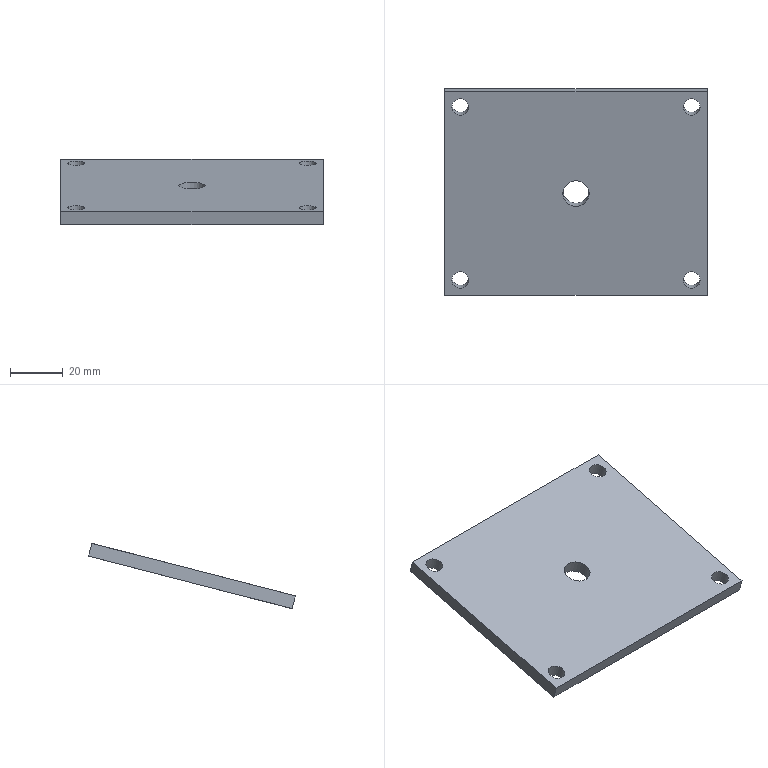Component | NX | SHIKONGGAI | 1 solid | 11 faces | box 100 x 78.71 x 24.84 mm | volume 38944 mm3 | plane 6 | cylinder 5 | commonest cylinder face diameters 6.5 x4 10 x1
STEP:
#1=CARTESIAN_POINT('',(0.,0.,0.));
#2=DIRECTION('',(0.,0.,1.));
#3=DIRECTION('',(1.,0.,0.));
#4=AXIS2_PLACEMENT_3D('',#1,#2,#3);
#5=CARTESIAN_POINT('',(-50.,133.02,11.412));
#6=VERTEX_POINT('',#5);
#7=CARTESIAN_POINT('',(-50.,55.56,-8.588));
#8=VERTEX_POINT('',#7);
#9=CARTESIAN_POINT('',(-50.,133.02,11.412));
#10=DIRECTION('',(0.,-0.9682,-0.25));
#11=VECTOR('',#10,1.);
#12=LINE('',#9,#11);
#13=CARTESIAN_POINT('',(-50.,131.77,16.253));
#14=DIRECTION('',(1.,0.,0.));
#15=DIRECTION('',(0.,0.25,-0.9682));
#16=AXIS2_PLACEMENT_3D('',#13,#14,#15);
#17=PLANE('',#16);
#18=CARTESIAN_POINT('',(5.,0.));
#19=DIRECTION('',(0.,-1.));
#20=VECTOR('',#19,1.);
#21=LINE('',#18,#20);
#22=(GEOMETRIC_REPRESENTATION_CONTEXT(2)PARAMETRIC_REPRESENTATION_CONTEXT()REPRESENTATION_CONTEXT('',''));
#23=DEFINITIONAL_REPRESENTATION('',(#21),#22);
#24=PCURVE('',#17,#23);
#25=CARTESIAN_POINT('',(44.,127.211,9.912));
#26=DIRECTION('',(0.,0.25,-0.9682));
#27=DIRECTION('',(-1.,0.,0.));
#28=AXIS2_PLACEMENT_3D('',#25,#26,#27);
#29=PLANE('',#28);
#30=CARTESIAN_POINT('',(94.,6.));
#31=DIRECTION('',(0.,-1.));
#32=VECTOR('',#31,1.);
#33=LINE('',#30,#32);
#34=(GEOMETRIC_REPRESENTATION_CONTEXT(2)PARAMETRIC_REPRESENTATION_CONTEXT()REPRESENTATION_CONTEXT('',''));
#35=DEFINITIONAL_REPRESENTATION('',(#33),#34);
#36=PCURVE('',#29,#35);
#37=SURFACE_CURVE('',#12,(#24,#36),.PCURVE_S1.);
#38=EDGE_CURVE('',#6,#8,#37,.T.);
#39=ORIENTED_EDGE('',*,*,#38,.T.);
#40=CARTESIAN_POINT('',(-50.,54.31,-3.747));
#41=VERTEX_POINT('',#40);
#42=CARTESIAN_POINT('',(-50.,54.31,-3.747));
#43=DIRECTION('',(0.,0.25,-0.9682));
#44=VECTOR('',#43,1.);
#45=LINE('',#42,#44);
#46=CARTESIAN_POINT('',(-0.,-80.));
#47=DIRECTION('',(1.,0.));
#48=VECTOR('',#47,1.);
#49=LINE('',#46,#48);
#50=(GEOMETRIC_REPRESENTATION_CONTEXT(2)PARAMETRIC_REPRESENTATION_CONTEXT()REPRESENTATION_CONTEXT('',''));
#51=DEFINITIONAL_REPRESENTATION('',(#49),#50);
#52=PCURVE('',#17,#51);
#53=CARTESIAN_POINT('',(-50.,54.31,-3.747));
#54=DIRECTION('',(0.,0.9682,0.25));
#55=DIRECTION('',(0.,-0.25,0.9682));
#56=AXIS2_PLACEMENT_3D('',#53,#54,#55);
#57=PLANE('',#56);
#58=CARTESIAN_POINT('',(0.,0.));
#59=DIRECTION('',(-1.,0.));
#60=VECTOR('',#59,1.);
#61=LINE('',#58,#60);
#62=(GEOMETRIC_REPRESENTATION_CONTEXT(2)PARAMETRIC_REPRESENTATION_CONTEXT()REPRESENTATION_CONTEXT('',''));
#63=DEFINITIONAL_REPRESENTATION('',(#61),#62);
#64=PCURVE('',#57,#63);
#65=SURFACE_CURVE('',#45,(#52,#64),.PCURVE_S1.);
#66=EDGE_CURVE('',#41,#8,#65,.T.);
#67=ORIENTED_EDGE('',*,*,#66,.F.);
#68=CARTESIAN_POINT('',(-50.,131.77,16.253));
#69=VERTEX_POINT('',#68);
#70=CARTESIAN_POINT('',(-50.,131.77,16.253));
#71=DIRECTION('',(0.,-0.9682,-0.25));
#72=VECTOR('',#71,1.);
#73=LINE('',#70,#72);
#74=CARTESIAN_POINT('',(0.,0.));
#75=DIRECTION('',(0.,-1.));
#76=VECTOR('',#75,1.);
#77=LINE('',#74,#76);
#78=(GEOMETRIC_REPRESENTATION_CONTEXT(2)PARAMETRIC_REPRESENTATION_CONTEXT()REPRESENTATION_CONTEXT('',''));
#79=DEFINITIONAL_REPRESENTATION('',(#77),#78);
#80=PCURVE('',#17,#79);
#81=CARTESIAN_POINT('',(44.,125.961,14.753));
#82=DIRECTION('',(0.,0.25,-0.9682));
#83=DIRECTION('',(-1.,0.,0.));
#84=AXIS2_PLACEMENT_3D('',#81,#82,#83);
#85=PLANE('',#84);
#86=CARTESIAN_POINT('',(94.,6.));
#87=DIRECTION('',(0.,-1.));
#88=VECTOR('',#87,1.);
#89=LINE('',#86,#88);
#90=(GEOMETRIC_REPRESENTATION_CONTEXT(2)PARAMETRIC_REPRESENTATION_CONTEXT()REPRESENTATION_CONTEXT('',''));
#91=DEFINITIONAL_REPRESENTATION('',(#89),#90);
#92=PCURVE('',#85,#91);
#93=SURFACE_CURVE('',#73,(#80,#92),.PCURVE_S1.);
#94=EDGE_CURVE('',#69,#41,#93,.T.);
#95=ORIENTED_EDGE('',*,*,#94,.F.);
#96=CARTESIAN_POINT('',(-50.,131.77,16.253));
#97=DIRECTION('',(0.,0.25,-0.9682));
#98=VECTOR('',#97,1.);
#99=LINE('',#96,#98);
#100=CARTESIAN_POINT('',(0.,0.));
#101=DIRECTION('',(1.,0.));
#102=VECTOR('',#101,1.);
#103=LINE('',#100,#102);
#104=(GEOMETRIC_REPRESENTATION_CONTEXT(2)PARAMETRIC_REPRESENTATION_CONTEXT()REPRESENTATION_CONTEXT('',''));
#105=DEFINITIONAL_REPRESENTATION('',(#103),#104);
#106=PCURVE('',#17,#105);
#107=CARTESIAN_POINT('',(50.,131.77,16.253));
#108=DIRECTION('',(0.,-0.9682,-0.25));
#109=DIRECTION('',(0.,0.25,-0.9682));
#110=AXIS2_PLACEMENT_3D('',#107,#108,#109);
#111=PLANE('',#110);
#112=CARTESIAN_POINT('',(0.,-100.));
#113=DIRECTION('',(1.,0.));
#114=VECTOR('',#113,1.);
#115=LINE('',#112,#114);
#116=(GEOMETRIC_REPRESENTATION_CONTEXT(2)PARAMETRIC_REPRESENTATION_CONTEXT()REPRESENTATION_CONTEXT('',''));
#117=DEFINITIONAL_REPRESENTATION('',(#115),#116);
#118=PCURVE('',#111,#117);
#119=SURFACE_CURVE('',#99,(#106,#118),.PCURVE_S1.);
#120=EDGE_CURVE('',#69,#6,#119,.T.);
#121=ORIENTED_EDGE('',*,*,#120,.T.);
#122=EDGE_LOOP('',(#39,#67,#95,#121));
#123=FACE_BOUND('',#122,.T.);
#124=ADVANCED_FACE('',(#123),#17,.F.);
#125=CARTESIAN_POINT('',(50.,55.56,-8.588));
#126=VERTEX_POINT('',#125);
#127=CARTESIAN_POINT('',(-50.,55.56,-8.588));
#128=DIRECTION('',(1.,0.,0.));
#129=VECTOR('',#128,1.);
#130=LINE('',#127,#129);
#131=CARTESIAN_POINT('',(-5.,0.));
#132=DIRECTION('',(0.,1.));
#133=VECTOR('',#132,1.);
#134=LINE('',#131,#133);
#135=(GEOMETRIC_REPRESENTATION_CONTEXT(2)PARAMETRIC_REPRESENTATION_CONTEXT()REPRESENTATION_CONTEXT('',''));
#136=DEFINITIONAL_REPRESENTATION('',(#134),#135);
#137=PCURVE('',#57,#136);
#138=CARTESIAN_POINT('',(94.,-74.));
#139=DIRECTION('',(-1.,0.));
#140=VECTOR('',#139,1.);
#141=LINE('',#138,#140);
#142=(GEOMETRIC_REPRESENTATION_CONTEXT(2)PARAMETRIC_REPRESENTATION_CONTEXT()REPRESENTATION_CONTEXT('',''));
#143=DEFINITIONAL_REPRESENTATION('',(#141),#142);
#144=PCURVE('',#29,#143);
#145=SURFACE_CURVE('',#130,(#137,#144),.PCURVE_S1.);
#146=EDGE_CURVE('',#8,#126,#145,.T.);
#147=ORIENTED_EDGE('',*,*,#146,.T.);
#148=CARTESIAN_POINT('',(50.,54.31,-3.747));
#149=VERTEX_POINT('',#148);
#150=CARTESIAN_POINT('',(50.,54.31,-3.747));
#151=DIRECTION('',(0.,0.25,-0.9682));
#152=VECTOR('',#151,1.);
#153=LINE('',#150,#152);
#154=CARTESIAN_POINT('',(0.,100.));
#155=DIRECTION('',(-1.,0.));
#156=VECTOR('',#155,1.);
#157=LINE('',#154,#156);
#158=(GEOMETRIC_REPRESENTATION_CONTEXT(2)PARAMETRIC_REPRESENTATION_CONTEXT()REPRESENTATION_CONTEXT('',''));
#159=DEFINITIONAL_REPRESENTATION('',(#157),#158);
#160=PCURVE('',#57,#159);
#161=CARTESIAN_POINT('',(50.,54.31,-3.747));
#162=DIRECTION('',(-1.,0.,0.));
#163=DIRECTION('',(0.,-0.25,0.9682));
#164=AXIS2_PLACEMENT_3D('',#161,#162,#163);
#165=PLANE('',#164);
#166=CARTESIAN_POINT('',(0.,0.));
#167=DIRECTION('',(-1.,0.));
#168=VECTOR('',#167,1.);
#169=LINE('',#166,#168);
#170=(GEOMETRIC_REPRESENTATION_CONTEXT(2)PARAMETRIC_REPRESENTATION_CONTEXT()REPRESENTATION_CONTEXT('',''));
#171=DEFINITIONAL_REPRESENTATION('',(#169),#170);
#172=PCURVE('',#165,#171);
#173=SURFACE_CURVE('',#153,(#160,#172),.PCURVE_S1.);
#174=EDGE_CURVE('',#149,#126,#173,.T.);
#175=ORIENTED_EDGE('',*,*,#174,.F.);
#176=CARTESIAN_POINT('',(-50.,54.31,-3.747));
#177=DIRECTION('',(1.,0.,0.));
#178=VECTOR('',#177,1.);
#179=LINE('',#176,#178);
#180=CARTESIAN_POINT('',(0.,0.));
#181=DIRECTION('',(0.,1.));
#182=VECTOR('',#181,1.);
#183=LINE('',#180,#182);
#184=(GEOMETRIC_REPRESENTATION_CONTEXT(2)PARAMETRIC_REPRESENTATION_CONTEXT()REPRESENTATION_CONTEXT('',''));
#185=DEFINITIONAL_REPRESENTATION('',(#183),#184);
#186=PCURVE('',#57,#185);
#187=CARTESIAN_POINT('',(94.,-74.));
#188=DIRECTION('',(-1.,0.));
#189=VECTOR('',#188,1.);
#190=LINE('',#187,#189);
#191=(GEOMETRIC_REPRESENTATION_CONTEXT(2)PARAMETRIC_REPRESENTATION_CONTEXT()REPRESENTATION_CONTEXT('',''));
#192=DEFINITIONAL_REPRESENTATION('',(#190),#191);
#193=PCURVE('',#85,#192);
#194=SURFACE_CURVE('',#179,(#186,#193),.PCURVE_S1.);
#195=EDGE_CURVE('',#41,#149,#194,.T.);
#196=ORIENTED_EDGE('',*,*,#195,.F.);
#197=ORIENTED_EDGE('',*,*,#66,.T.);
#198=EDGE_LOOP('',(#147,#175,#196,#197));
#199=FACE_BOUND('',#198,.T.);
#200=ADVANCED_FACE('',(#199),#57,.F.);
#201=CARTESIAN_POINT('',(50.,133.02,11.412));
#202=VERTEX_POINT('',#201);
#203=CARTESIAN_POINT('',(50.,55.56,-8.588));
#204=DIRECTION('',(0.,0.9682,0.25));
#205=VECTOR('',#204,1.);
#206=LINE('',#203,#205);
#207=CARTESIAN_POINT('',(-5.,0.));
#208=DIRECTION('',(0.,1.));
#209=VECTOR('',#208,1.);
#210=LINE('',#207,#209);
#211=(GEOMETRIC_REPRESENTATION_CONTEXT(2)PARAMETRIC_REPRESENTATION_CONTEXT()REPRESENTATION_CONTEXT('',''));
#212=DEFINITIONAL_REPRESENTATION('',(#210),#211);
#213=PCURVE('',#165,#212);
#214=CARTESIAN_POINT('',(-6.,-74.));
#215=DIRECTION('',(0.,1.));
#216=VECTOR('',#215,1.);
#217=LINE('',#214,#216);
#218=(GEOMETRIC_REPRESENTATION_CONTEXT(2)PARAMETRIC_REPRESENTATION_CONTEXT()REPRESENTATION_CONTEXT('',''));
#219=DEFINITIONAL_REPRESENTATION('',(#217),#218);
#220=PCURVE('',#29,#219);
#221=SURFACE_CURVE('',#206,(#213,#220),.PCURVE_S1.);
#222=EDGE_CURVE('',#126,#202,#221,.T.);
#223=ORIENTED_EDGE('',*,*,#222,.T.);
#224=CARTESIAN_POINT('',(50.,131.77,16.253));
#225=VERTEX_POINT('',#224);
#226=CARTESIAN_POINT('',(50.,131.77,16.253));
#227=DIRECTION('',(0.,0.25,-0.9682));
#228=VECTOR('',#227,1.);
#229=LINE('',#226,#228);
#230=CARTESIAN_POINT('',(-0.,80.));
#231=DIRECTION('',(-1.,0.));
#232=VECTOR('',#231,1.);
#233=LINE('',#230,#232);
#234=(GEOMETRIC_REPRESENTATION_CONTEXT(2)PARAMETRIC_REPRESENTATION_CONTEXT()REPRESENTATION_CONTEXT('',''));
#235=DEFINITIONAL_REPRESENTATION('',(#233),#234);
#236=PCURVE('',#165,#235);
#237=CARTESIAN_POINT('',(0.,0.));
#238=DIRECTION('',(1.,0.));
#239=VECTOR('',#238,1.);
#240=LINE('',#237,#239);
#241=(GEOMETRIC_REPRESENTATION_CONTEXT(2)PARAMETRIC_REPRESENTATION_CONTEXT()REPRESENTATION_CONTEXT('',''));
#242=DEFINITIONAL_REPRESENTATION('',(#240),#241);
#243=PCURVE('',#111,#242);
#244=SURFACE_CURVE('',#229,(#236,#243),.PCURVE_S1.);
#245=EDGE_CURVE('',#225,#202,#244,.T.);
#246=ORIENTED_EDGE('',*,*,#245,.F.);
#247=CARTESIAN_POINT('',(50.,54.31,-3.747));
#248=DIRECTION('',(0.,0.9682,0.25));
#249=VECTOR('',#248,1.);
#250=LINE('',#247,#249);
#251=CARTESIAN_POINT('',(0.,0.));
#252=DIRECTION('',(0.,1.));
#253=VECTOR('',#252,1.);
#254=LINE('',#251,#253);
#255=(GEOMETRIC_REPRESENTATION_CONTEXT(2)PARAMETRIC_REPRESENTATION_CONTEXT()REPRESENTATION_CONTEXT('',''));
#256=DEFINITIONAL_REPRESENTATION('',(#254),#255);
#257=PCURVE('',#165,#256);
#258=CARTESIAN_POINT('',(-6.,-74.));
#259=DIRECTION('',(0.,1.));
#260=VECTOR('',#259,1.);
#261=LINE('',#258,#260);
#262=(GEOMETRIC_REPRESENTATION_CONTEXT(2)PARAMETRIC_REPRESENTATION_CONTEXT()REPRESENTATION_CONTEXT('',''));
#263=DEFINITIONAL_REPRESENTATION('',(#261),#262);
#264=PCURVE('',#85,#263);
#265=SURFACE_CURVE('',#250,(#257,#264),.PCURVE_S1.);
#266=EDGE_CURVE('',#149,#225,#265,.T.);
#267=ORIENTED_EDGE('',*,*,#266,.F.);
#268=ORIENTED_EDGE('',*,*,#174,.T.);
#269=EDGE_LOOP('',(#223,#246,#267,#268));
#270=FACE_BOUND('',#269,.T.);
#271=ADVANCED_FACE('',(#270),#165,.F.);
#272=CARTESIAN_POINT('',(-40.75,125.961,14.753));
#273=VERTEX_POINT('',#272);
#274=CARTESIAN_POINT('',(-44.,125.961,14.753));
#275=DIRECTION('',(0.,-0.25,0.9682));
#276=DIRECTION('',(1.,0.,0.));
#277=AXIS2_PLACEMENT_3D('',#274,#275,#276);
#278=CIRCLE('',#277,3.25);
#279=CARTESIAN_POINT('',(-44.,125.961,14.753));
#280=DIRECTION('',(0.,0.25,-0.9682));
#281=DIRECTION('',(-1.,0.,0.));
#282=AXIS2_PLACEMENT_3D('',#279,#280,#281);
#283=CYLINDRICAL_SURFACE('',#282,3.25);
#284=CARTESIAN_POINT('',(9.425,0.));
#285=DIRECTION('',(-1.,0.));
#286=VECTOR('',#285,1.);
#287=LINE('',#284,#286);
#288=(GEOMETRIC_REPRESENTATION_CONTEXT(2)PARAMETRIC_REPRESENTATION_CONTEXT()REPRESENTATION_CONTEXT('',''));
#289=DEFINITIONAL_REPRESENTATION('',(#287),#288);
#290=PCURVE('',#283,#289);
#291=CARTESIAN_POINT('',(84.75,0.));
#292=CARTESIAN_POINT('',(84.75,5.629));
#293=CARTESIAN_POINT('',(89.625,2.815));
#294=CARTESIAN_POINT('',(94.5,0.));
#295=CARTESIAN_POINT('',(89.625,-2.815));
#296=CARTESIAN_POINT('',(84.75,-5.629));
#297=CARTESIAN_POINT('',(84.75,0.));
#298=(BOUNDED_CURVE()B_SPLINE_CURVE(2,(#291,#292,#293,#294,#295,#296,#297),.UNSPECIFIED.,.T.,.F.)B_SPLINE_CURVE_WITH_KNOTS((1,2,2,2,2,1),(-2.094,0.,2.094,4.189,6.283,8.378),.UNSPECIFIED.)CURVE()GEOMETRIC_REPRESENTATION_ITEM()RATIONAL_B_SPLINE_CURVE((1.,0.5,1.,0.5,1.,0.5,1.))REPRESENTATION_ITEM(''));
#299=(GEOMETRIC_REPRESENTATION_CONTEXT(2)PARAMETRIC_REPRESENTATION_CONTEXT()REPRESENTATION_CONTEXT('',''));
#300=DEFINITIONAL_REPRESENTATION('',(#298),#299);
#301=PCURVE('',#85,#300);
#302=SURFACE_CURVE('',#278,(#290,#301),.PCURVE_S1.);
#303=EDGE_CURVE('',#273,#273,#302,.T.);
#304=ORIENTED_EDGE('',*,*,#303,.F.);
#305=CARTESIAN_POINT('',(-40.75,127.211,9.912));
#306=VERTEX_POINT('',#305);
#307=CARTESIAN_POINT('',(-40.75,125.961,14.753));
#308=CARTESIAN_POINT('',(-40.75,127.211,9.912));
#309=B_SPLINE_CURVE_WITH_KNOTS('',1,(#307,#308),.UNSPECIFIED.,.F.,.F.,(2,2),(0.,5.),.PIECEWISE_BEZIER_KNOTS.);
#310=CARTESIAN_POINT('',(9.425,0.));
#311=DIRECTION('',(0.,1.));
#312=VECTOR('',#311,1.);
#313=LINE('',#310,#312);
#314=(GEOMETRIC_REPRESENTATION_CONTEXT(2)PARAMETRIC_REPRESENTATION_CONTEXT()REPRESENTATION_CONTEXT('',''));
#315=DEFINITIONAL_REPRESENTATION('',(#313),#314);
#316=PCURVE('',#283,#315);
#317=CARTESIAN_POINT('',(3.142,0.));
#318=DIRECTION('',(0.,1.));
#319=VECTOR('',#318,1.);
#320=LINE('',#317,#319);
#321=(GEOMETRIC_REPRESENTATION_CONTEXT(2)PARAMETRIC_REPRESENTATION_CONTEXT()REPRESENTATION_CONTEXT('',''));
#322=DEFINITIONAL_REPRESENTATION('',(#320),#321);
#323=PCURVE('',#283,#322);
#324=SEAM_CURVE('',#309,(#316,#323),.PCURVE_S1.);
#325=EDGE_CURVE('',#273,#306,#324,.T.);
#326=ORIENTED_EDGE('',*,*,#325,.T.);
#327=CARTESIAN_POINT('',(-44.,127.211,9.912));
#328=DIRECTION('',(0.,-0.25,0.9682));
#329=DIRECTION('',(1.,0.,0.));
#330=AXIS2_PLACEMENT_3D('',#327,#328,#329);
#331=CIRCLE('',#330,3.25);
#332=CARTESIAN_POINT('',(9.425,5.));
#333=DIRECTION('',(-1.,0.));
#334=VECTOR('',#333,1.);
#335=LINE('',#332,#334);
#336=(GEOMETRIC_REPRESENTATION_CONTEXT(2)PARAMETRIC_REPRESENTATION_CONTEXT()REPRESENTATION_CONTEXT('',''));
#337=DEFINITIONAL_REPRESENTATION('',(#335),#336);
#338=PCURVE('',#283,#337);
#339=CARTESIAN_POINT('',(84.75,0.));
#340=CARTESIAN_POINT('',(84.75,5.629));
#341=CARTESIAN_POINT('',(89.625,2.815));
#342=CARTESIAN_POINT('',(94.5,0.));
#343=CARTESIAN_POINT('',(89.625,-2.815));
#344=CARTESIAN_POINT('',(84.75,-5.629));
#345=CARTESIAN_POINT('',(84.75,0.));
#346=(BOUNDED_CURVE()B_SPLINE_CURVE(2,(#339,#340,#341,#342,#343,#344,#345),.UNSPECIFIED.,.T.,.F.)B_SPLINE_CURVE_WITH_KNOTS((1,2,2,2,2,1),(-2.094,0.,2.094,4.189,6.283,8.378),.UNSPECIFIED.)CURVE()GEOMETRIC_REPRESENTATION_ITEM()RATIONAL_B_SPLINE_CURVE((1.,0.5,1.,0.5,1.,0.5,1.))REPRESENTATION_ITEM(''));
#347=(GEOMETRIC_REPRESENTATION_CONTEXT(2)PARAMETRIC_REPRESENTATION_CONTEXT()REPRESENTATION_CONTEXT('',''));
#348=DEFINITIONAL_REPRESENTATION('',(#346),#347);
#349=PCURVE('',#29,#348);
#350=SURFACE_CURVE('',#331,(#338,#349),.PCURVE_S1.);
#351=EDGE_CURVE('',#306,#306,#350,.T.);
#352=ORIENTED_EDGE('',*,*,#351,.T.);
#353=ORIENTED_EDGE('',*,*,#325,.F.);
#354=EDGE_LOOP('',(#304,#326,#352,#353));
#355=FACE_BOUND('',#354,.F.);
#356=ADVANCED_FACE('',(#355),#283,.F.);
#357=CARTESIAN_POINT('',(40.75,60.12,-2.247));
#358=VERTEX_POINT('',#357);
#359=CARTESIAN_POINT('',(44.,60.12,-2.247));
#360=DIRECTION('',(0.,-0.25,0.9682));
#361=DIRECTION('',(-1.,0.,0.));
#362=AXIS2_PLACEMENT_3D('',#359,#360,#361);
#363=CIRCLE('',#362,3.25);
#364=CARTESIAN_POINT('',(44.,60.12,-2.247));
#365=DIRECTION('',(0.,0.25,-0.9682));
#366=DIRECTION('',(-1.,0.,0.));
#367=AXIS2_PLACEMENT_3D('',#364,#365,#366);
#368=CYLINDRICAL_SURFACE('',#367,3.25);
#369=CARTESIAN_POINT('',(6.283,0.));
#370=DIRECTION('',(-1.,0.));
#371=VECTOR('',#370,1.);
#372=LINE('',#369,#371);
#373=(GEOMETRIC_REPRESENTATION_CONTEXT(2)PARAMETRIC_REPRESENTATION_CONTEXT()REPRESENTATION_CONTEXT('',''));
#374=DEFINITIONAL_REPRESENTATION('',(#372),#373);
#375=PCURVE('',#368,#374);
#376=CARTESIAN_POINT('',(3.25,-68.));
#377=CARTESIAN_POINT('',(3.25,-73.629));
#378=CARTESIAN_POINT('',(-1.625,-70.815));
#379=CARTESIAN_POINT('',(-6.5,-68.));
#380=CARTESIAN_POINT('',(-1.625,-65.185));
#381=CARTESIAN_POINT('',(3.25,-62.371));
#382=CARTESIAN_POINT('',(3.25,-68.));
#383=(BOUNDED_CURVE()B_SPLINE_CURVE(2,(#376,#377,#378,#379,#380,#381,#382),.UNSPECIFIED.,.T.,.F.)B_SPLINE_CURVE_WITH_KNOTS((1,2,2,2,2,1),(-2.094,0.,2.094,4.189,6.283,8.378),.UNSPECIFIED.)CURVE()GEOMETRIC_REPRESENTATION_ITEM()RATIONAL_B_SPLINE_CURVE((1.,0.5,1.,0.5,1.,0.5,1.))REPRESENTATION_ITEM(''));
#384=(GEOMETRIC_REPRESENTATION_CONTEXT(2)PARAMETRIC_REPRESENTATION_CONTEXT()REPRESENTATION_CONTEXT('',''));
#385=DEFINITIONAL_REPRESENTATION('',(#383),#384);
#386=PCURVE('',#85,#385);
#387=SURFACE_CURVE('',#363,(#375,#386),.PCURVE_S1.);
#388=EDGE_CURVE('',#358,#358,#387,.T.);
#389=ORIENTED_EDGE('',*,*,#388,.F.);
#390=CARTESIAN_POINT('',(40.75,61.37,-7.088));
#391=VERTEX_POINT('',#390);
#392=CARTESIAN_POINT('',(40.75,60.12,-2.247));
#393=CARTESIAN_POINT('',(40.75,61.37,-7.088));
#394=B_SPLINE_CURVE_WITH_KNOTS('',1,(#392,#393),.UNSPECIFIED.,.F.,.F.,(2,2),(0.,5.),.PIECEWISE_BEZIER_KNOTS.);
#395=CARTESIAN_POINT('',(6.283,0.));
#396=DIRECTION('',(0.,1.));
#397=VECTOR('',#396,1.);
#398=LINE('',#395,#397);
#399=(GEOMETRIC_REPRESENTATION_CONTEXT(2)PARAMETRIC_REPRESENTATION_CONTEXT()REPRESENTATION_CONTEXT('',''));
#400=DEFINITIONAL_REPRESENTATION('',(#398),#399);
#401=PCURVE('',#368,#400);
#402=CARTESIAN_POINT('',(0.,0.));
#403=DIRECTION('',(0.,1.));
#404=VECTOR('',#403,1.);
#405=LINE('',#402,#404);
#406=(GEOMETRIC_REPRESENTATION_CONTEXT(2)PARAMETRIC_REPRESENTATION_CONTEXT()REPRESENTATION_CONTEXT('',''));
#407=DEFINITIONAL_REPRESENTATION('',(#405),#406);
#408=PCURVE('',#368,#407);
#409=SEAM_CURVE('',#394,(#401,#408),.PCURVE_S1.);
#410=EDGE_CURVE('',#358,#391,#409,.T.);
#411=ORIENTED_EDGE('',*,*,#410,.T.);
#412=CARTESIAN_POINT('',(44.,61.37,-7.088));
#413=DIRECTION('',(0.,-0.25,0.9682));
#414=DIRECTION('',(-1.,0.,0.));
#415=AXIS2_PLACEMENT_3D('',#412,#413,#414);
#416=CIRCLE('',#415,3.25);
#417=CARTESIAN_POINT('',(6.283,5.));
#418=DIRECTION('',(-1.,0.));
#419=VECTOR('',#418,1.);
#420=LINE('',#417,#419);
#421=(GEOMETRIC_REPRESENTATION_CONTEXT(2)PARAMETRIC_REPRESENTATION_CONTEXT()REPRESENTATION_CONTEXT('',''));
#422=DEFINITIONAL_REPRESENTATION('',(#420),#421);
#423=PCURVE('',#368,#422);
#424=CARTESIAN_POINT('',(3.25,-68.));
#425=CARTESIAN_POINT('',(3.25,-73.629));
#426=CARTESIAN_POINT('',(-1.625,-70.815));
#427=CARTESIAN_POINT('',(-6.5,-68.));
#428=CARTESIAN_POINT('',(-1.625,-65.185));
#429=CARTESIAN_POINT('',(3.25,-62.371));
#430=CARTESIAN_POINT('',(3.25,-68.));
#431=(BOUNDED_CURVE()B_SPLINE_CURVE(2,(#424,#425,#426,#427,#428,#429,#430),.UNSPECIFIED.,.T.,.F.)B_SPLINE_CURVE_WITH_KNOTS((1,2,2,2,2,1),(-2.094,0.,2.094,4.189,6.283,8.378),.UNSPECIFIED.)CURVE()GEOMETRIC_REPRESENTATION_ITEM()RATIONAL_B_SPLINE_CURVE((1.,0.5,1.,0.5,1.,0.5,1.))REPRESENTATION_ITEM(''));
#432=(GEOMETRIC_REPRESENTATION_CONTEXT(2)PARAMETRIC_REPRESENTATION_CONTEXT()REPRESENTATION_CONTEXT('',''));
#433=DEFINITIONAL_REPRESENTATION('',(#431),#432);
#434=PCURVE('',#29,#433);
#435=SURFACE_CURVE('',#416,(#423,#434),.PCURVE_S1.);
#436=EDGE_CURVE('',#391,#391,#435,.T.);
#437=ORIENTED_EDGE('',*,*,#436,.T.);
#438=ORIENTED_EDGE('',*,*,#410,.F.);
#439=EDGE_LOOP('',(#389,#411,#437,#438));
#440=FACE_BOUND('',#439,.F.);
#441=ADVANCED_FACE('',(#440),#368,.F.);
#442=CARTESIAN_POINT('',(40.75,125.961,14.753));
#443=VERTEX_POINT('',#442);
#444=CARTESIAN_POINT('',(44.,125.961,14.753));
#445=DIRECTION('',(0.,0.25,-0.9682));
#446=DIRECTION('',(-1.,0.,0.));
#447=AXIS2_PLACEMENT_3D('',#444,#445,#446);
#448=CIRCLE('',#447,3.25);
#449=CARTESIAN_POINT('',(44.,125.961,14.753));
#450=DIRECTION('',(0.,0.25,-0.9682));
#451=DIRECTION('',(-1.,0.,0.));
#452=AXIS2_PLACEMENT_3D('',#449,#450,#451);
#453=CYLINDRICAL_SURFACE('',#452,3.25);
#454=CARTESIAN_POINT('',(0.,0.));
#455=DIRECTION('',(1.,0.));
#456=VECTOR('',#455,1.);
#457=LINE('',#454,#456);
#458=(GEOMETRIC_REPRESENTATION_CONTEXT(2)PARAMETRIC_REPRESENTATION_CONTEXT()REPRESENTATION_CONTEXT('',''));
#459=DEFINITIONAL_REPRESENTATION('',(#457),#458);
#460=PCURVE('',#453,#459);
#461=CARTESIAN_POINT('',(0.,0.));
#462=DIRECTION('',(1.,0.));
#463=AXIS2_PLACEMENT_2D('',#461,#462);
#464=CIRCLE('',#463,3.25);
#465=(GEOMETRIC_REPRESENTATION_CONTEXT(2)PARAMETRIC_REPRESENTATION_CONTEXT()REPRESENTATION_CONTEXT('',''));
#466=DEFINITIONAL_REPRESENTATION('',(#464),#465);
#467=PCURVE('',#85,#466);
#468=SURFACE_CURVE('',#448,(#460,#467),.PCURVE_S1.);
#469=EDGE_CURVE('',#443,#443,#468,.T.);
#470=ORIENTED_EDGE('',*,*,#469,.T.);
#471=CARTESIAN_POINT('',(40.75,127.211,9.912));
#472=VERTEX_POINT('',#471);
#473=CARTESIAN_POINT('',(40.75,125.961,14.753));
#474=CARTESIAN_POINT('',(40.75,127.211,9.912));
#475=B_SPLINE_CURVE_WITH_KNOTS('',1,(#473,#474),.UNSPECIFIED.,.F.,.F.,(2,2),(0.,5.),.PIECEWISE_BEZIER_KNOTS.);
#476=CARTESIAN_POINT('',(6.283,0.));
#477=DIRECTION('',(0.,1.));
#478=VECTOR('',#477,1.);
#479=LINE('',#476,#478);
#480=(GEOMETRIC_REPRESENTATION_CONTEXT(2)PARAMETRIC_REPRESENTATION_CONTEXT()REPRESENTATION_CONTEXT('',''));
#481=DEFINITIONAL_REPRESENTATION('',(#479),#480);
#482=PCURVE('',#453,#481);
#483=CARTESIAN_POINT('',(0.,0.));
#484=DIRECTION('',(0.,1.));
#485=VECTOR('',#484,1.);
#486=LINE('',#483,#485);
#487=(GEOMETRIC_REPRESENTATION_CONTEXT(2)PARAMETRIC_REPRESENTATION_CONTEXT()REPRESENTATION_CONTEXT('',''));
#488=DEFINITIONAL_REPRESENTATION('',(#486),#487);
#489=PCURVE('',#453,#488);
#490=SEAM_CURVE('',#475,(#482,#489),.PCURVE_S1.);
#491=EDGE_CURVE('',#443,#472,#490,.T.);
#492=ORIENTED_EDGE('',*,*,#491,.T.);
#493=CARTESIAN_POINT('',(44.,127.211,9.912));
#494=DIRECTION('',(0.,0.25,-0.9682));
#495=DIRECTION('',(-1.,0.,0.));
#496=AXIS2_PLACEMENT_3D('',#493,#494,#495);
#497=CIRCLE('',#496,3.25);
#498=CARTESIAN_POINT('',(0.,5.));
#499=DIRECTION('',(1.,0.));
#500=VECTOR('',#499,1.);
#501=LINE('',#498,#500);
#502=(GEOMETRIC_REPRESENTATION_CONTEXT(2)PARAMETRIC_REPRESENTATION_CONTEXT()REPRESENTATION_CONTEXT('',''));
#503=DEFINITIONAL_REPRESENTATION('',(#501),#502);
#504=PCURVE('',#453,#503);
#505=CARTESIAN_POINT('',(0.,0.));
#506=DIRECTION('',(1.,0.));
#507=AXIS2_PLACEMENT_2D('',#505,#506);
#508=CIRCLE('',#507,3.25);
#509=(GEOMETRIC_REPRESENTATION_CONTEXT(2)PARAMETRIC_REPRESENTATION_CONTEXT()REPRESENTATION_CONTEXT('',''));
#510=DEFINITIONAL_REPRESENTATION('',(#508),#509);
#511=PCURVE('',#29,#510);
#512=SURFACE_CURVE('',#497,(#504,#511),.PCURVE_S1.);
#513=EDGE_CURVE('',#472,#472,#512,.T.);
#514=ORIENTED_EDGE('',*,*,#513,.F.);
#515=ORIENTED_EDGE('',*,*,#491,.F.);
#516=EDGE_LOOP('',(#470,#492,#514,#515));
#517=FACE_BOUND('',#516,.F.);
#518=ADVANCED_FACE('',(#517),#453,.F.);
#519=CARTESIAN_POINT('',(50.,133.02,11.412));
#520=DIRECTION('',(-1.,0.,0.));
#521=VECTOR('',#520,1.);
#522=LINE('',#519,#521);
#523=CARTESIAN_POINT('',(5.,0.));
#524=DIRECTION('',(0.,-1.));
#525=VECTOR('',#524,1.);
#526=LINE('',#523,#525);
#527=(GEOMETRIC_REPRESENTATION_CONTEXT(2)PARAMETRIC_REPRESENTATION_CONTEXT()REPRESENTATION_CONTEXT('',''));
#528=DEFINITIONAL_REPRESENTATION('',(#526),#527);
#529=PCURVE('',#111,#528);
#530=CARTESIAN_POINT('',(-6.,6.));
#531=DIRECTION('',(1.,0.));
#532=VECTOR('',#531,1.);
#533=LINE('',#530,#532);
#534=(GEOMETRIC_REPRESENTATION_CONTEXT(2)PARAMETRIC_REPRESENTATION_CONTEXT()REPRESENTATION_CONTEXT('',''));
#535=DEFINITIONAL_REPRESENTATION('',(#533),#534);
#536=PCURVE('',#29,#535);
#537=SURFACE_CURVE('',#522,(#529,#536),.PCURVE_S1.);
#538=EDGE_CURVE('',#202,#6,#537,.T.);
#539=ORIENTED_EDGE('',*,*,#538,.T.);
#540=ORIENTED_EDGE('',*,*,#120,.F.);
#541=CARTESIAN_POINT('',(50.,131.77,16.253));
#542=DIRECTION('',(-1.,0.,0.));
#543=VECTOR('',#542,1.);
#544=LINE('',#541,#543);
#545=CARTESIAN_POINT('',(0.,0.));
#546=DIRECTION('',(0.,-1.));
#547=VECTOR('',#546,1.);
#548=LINE('',#545,#547);
#549=(GEOMETRIC_REPRESENTATION_CONTEXT(2)PARAMETRIC_REPRESENTATION_CONTEXT()REPRESENTATION_CONTEXT('',''));
#550=DEFINITIONAL_REPRESENTATION('',(#548),#549);
#551=PCURVE('',#111,#550);
#552=CARTESIAN_POINT('',(-6.,6.));
#553=DIRECTION('',(1.,0.));
#554=VECTOR('',#553,1.);
#555=LINE('',#552,#554);
#556=(GEOMETRIC_REPRESENTATION_CONTEXT(2)PARAMETRIC_REPRESENTATION_CONTEXT()REPRESENTATION_CONTEXT('',''));
#557=DEFINITIONAL_REPRESENTATION('',(#555),#556);
#558=PCURVE('',#85,#557);
#559=SURFACE_CURVE('',#544,(#551,#558),.PCURVE_S1.);
#560=EDGE_CURVE('',#225,#69,#559,.T.);
#561=ORIENTED_EDGE('',*,*,#560,.F.);
#562=ORIENTED_EDGE('',*,*,#245,.T.);
#563=EDGE_LOOP('',(#539,#540,#561,#562));
#564=FACE_BOUND('',#563,.T.);
#565=ADVANCED_FACE('',(#564),#111,.F.);
#566=CARTESIAN_POINT('',(-40.75,60.12,-2.247));
#567=VERTEX_POINT('',#566);
#568=CARTESIAN_POINT('',(-44.,60.12,-2.247));
#569=DIRECTION('',(0.,0.25,-0.9682));
#570=DIRECTION('',(1.,0.,0.));
#571=AXIS2_PLACEMENT_3D('',#568,#569,#570);
#572=CIRCLE('',#571,3.25);
#573=CARTESIAN_POINT('',(-44.,60.12,-2.247));
#574=DIRECTION('',(0.,0.25,-0.9682));
#575=DIRECTION('',(-1.,0.,0.));
#576=AXIS2_PLACEMENT_3D('',#573,#574,#575);
#577=CYLINDRICAL_SURFACE('',#576,3.25);
#578=CARTESIAN_POINT('',(3.142,0.));
#579=DIRECTION('',(1.,0.));
#580=VECTOR('',#579,1.);
#581=LINE('',#578,#580);
#582=(GEOMETRIC_REPRESENTATION_CONTEXT(2)PARAMETRIC_REPRESENTATION_CONTEXT()REPRESENTATION_CONTEXT('',''));
#583=DEFINITIONAL_REPRESENTATION('',(#581),#582);
#584=PCURVE('',#577,#583);
#585=CARTESIAN_POINT('',(88.,-68.));
#586=DIRECTION('',(-1.,0.));
#587=AXIS2_PLACEMENT_2D('',#585,#586);
#588=CIRCLE('',#587,3.25);
#589=(GEOMETRIC_REPRESENTATION_CONTEXT(2)PARAMETRIC_REPRESENTATION_CONTEXT()REPRESENTATION_CONTEXT('',''));
#590=DEFINITIONAL_REPRESENTATION('',(#588),#589);
#591=PCURVE('',#85,#590);
#592=SURFACE_CURVE('',#572,(#584,#591),.PCURVE_S1.);
#593=EDGE_CURVE('',#567,#567,#592,.T.);
#594=ORIENTED_EDGE('',*,*,#593,.T.);
#595=CARTESIAN_POINT('',(-40.75,61.37,-7.088));
#596=VERTEX_POINT('',#595);
#597=CARTESIAN_POINT('',(-40.75,60.12,-2.247));
#598=CARTESIAN_POINT('',(-40.75,61.37,-7.088));
#599=B_SPLINE_CURVE_WITH_KNOTS('',1,(#597,#598),.UNSPECIFIED.,.F.,.F.,(2,2),(0.,5.),.PIECEWISE_BEZIER_KNOTS.);
#600=CARTESIAN_POINT('',(9.425,0.));
#601=DIRECTION('',(0.,1.));
#602=VECTOR('',#601,1.);
#603=LINE('',#600,#602);
#604=(GEOMETRIC_REPRESENTATION_CONTEXT(2)PARAMETRIC_REPRESENTATION_CONTEXT()REPRESENTATION_CONTEXT('',''));
#605=DEFINITIONAL_REPRESENTATION('',(#603),#604);
#606=PCURVE('',#577,#605);
#607=CARTESIAN_POINT('',(3.142,0.));
#608=DIRECTION('',(0.,1.));
#609=VECTOR('',#608,1.);
#610=LINE('',#607,#609);
#611=(GEOMETRIC_REPRESENTATION_CONTEXT(2)PARAMETRIC_REPRESENTATION_CONTEXT()REPRESENTATION_CONTEXT('',''));
#612=DEFINITIONAL_REPRESENTATION('',(#610),#611);
#613=PCURVE('',#577,#612);
#614=SEAM_CURVE('',#599,(#606,#613),.PCURVE_S1.);
#615=EDGE_CURVE('',#567,#596,#614,.T.);
#616=ORIENTED_EDGE('',*,*,#615,.T.);
#617=CARTESIAN_POINT('',(-44.,61.37,-7.088));
#618=DIRECTION('',(0.,0.25,-0.9682));
#619=DIRECTION('',(1.,0.,0.));
#620=AXIS2_PLACEMENT_3D('',#617,#618,#619);
#621=CIRCLE('',#620,3.25);
#622=CARTESIAN_POINT('',(3.142,5.));
#623=DIRECTION('',(1.,0.));
#624=VECTOR('',#623,1.);
#625=LINE('',#622,#624);
#626=(GEOMETRIC_REPRESENTATION_CONTEXT(2)PARAMETRIC_REPRESENTATION_CONTEXT()REPRESENTATION_CONTEXT('',''));
#627=DEFINITIONAL_REPRESENTATION('',(#625),#626);
#628=PCURVE('',#577,#627);
#629=CARTESIAN_POINT('',(88.,-68.));
#630=DIRECTION('',(-1.,0.));
#631=AXIS2_PLACEMENT_2D('',#629,#630);
#632=CIRCLE('',#631,3.25);
#633=(GEOMETRIC_REPRESENTATION_CONTEXT(2)PARAMETRIC_REPRESENTATION_CONTEXT()REPRESENTATION_CONTEXT('',''));
#634=DEFINITIONAL_REPRESENTATION('',(#632),#633);
#635=PCURVE('',#29,#634);
#636=SURFACE_CURVE('',#621,(#628,#635),.PCURVE_S1.);
#637=EDGE_CURVE('',#596,#596,#636,.T.);
#638=ORIENTED_EDGE('',*,*,#637,.F.);
#639=ORIENTED_EDGE('',*,*,#615,.F.);
#640=EDGE_LOOP('',(#594,#616,#638,#639));
#641=FACE_BOUND('',#640,.F.);
#642=ADVANCED_FACE('',(#641),#577,.F.);
#643=CARTESIAN_POINT('',(-5.,93.04,6.253));
#644=VERTEX_POINT('',#643);
#645=CARTESIAN_POINT('',(5.,93.04,6.253));
#646=VERTEX_POINT('',#645);
#647=CARTESIAN_POINT('',(0.,93.04,6.253));
#648=DIRECTION('',(0.,0.25,-0.9682));
#649=DIRECTION('',(-1.,0.,0.));
#650=AXIS2_PLACEMENT_3D('',#647,#648,#649);
#651=CIRCLE('',#650,5.);
#652=CARTESIAN_POINT('',(44.,-34.));
#653=DIRECTION('',(1.,0.));
#654=AXIS2_PLACEMENT_2D('',#652,#653);
#655=CIRCLE('',#654,5.);
#656=(GEOMETRIC_REPRESENTATION_CONTEXT(2)PARAMETRIC_REPRESENTATION_CONTEXT()REPRESENTATION_CONTEXT('',''));
#657=DEFINITIONAL_REPRESENTATION('',(#655),#656);
#658=PCURVE('',#85,#657);
#659=CARTESIAN_POINT('',(0.,94.29,1.412));
#660=DIRECTION('',(0.,-0.25,0.9682));
#661=DIRECTION('',(1.,0.,0.));
#662=AXIS2_PLACEMENT_3D('',#659,#660,#661);
#663=CYLINDRICAL_SURFACE('',#662,5.);
#664=CARTESIAN_POINT('',(3.142,5.));
#665=DIRECTION('',(-1.,0.));
#666=VECTOR('',#665,1.);
#667=LINE('',#664,#666);
#668=(GEOMETRIC_REPRESENTATION_CONTEXT(2)PARAMETRIC_REPRESENTATION_CONTEXT()REPRESENTATION_CONTEXT('',''));
#669=DEFINITIONAL_REPRESENTATION('',(#667),#668);
#670=PCURVE('',#663,#669);
#671=SURFACE_CURVE('',#651,(#658,#670),.PCURVE_S1.);
#672=EDGE_CURVE('',#644,#646,#671,.T.);
#673=ORIENTED_EDGE('',*,*,#672,.T.);
#674=CARTESIAN_POINT('',(0.,93.04,6.253));
#675=DIRECTION('',(0.,0.25,-0.9682));
#676=DIRECTION('',(-1.,0.,0.));
#677=AXIS2_PLACEMENT_3D('',#674,#675,#676);
#678=CIRCLE('',#677,5.);
#679=CARTESIAN_POINT('',(44.,-34.));
#680=DIRECTION('',(1.,0.));
#681=AXIS2_PLACEMENT_2D('',#679,#680);
#682=CIRCLE('',#681,5.);
#683=(GEOMETRIC_REPRESENTATION_CONTEXT(2)PARAMETRIC_REPRESENTATION_CONTEXT()REPRESENTATION_CONTEXT('',''));
#684=DEFINITIONAL_REPRESENTATION('',(#682),#683);
#685=PCURVE('',#85,#684);
#686=CARTESIAN_POINT('',(9.425,5.));
#687=DIRECTION('',(-1.,0.));
#688=VECTOR('',#687,1.);
#689=LINE('',#686,#688);
#690=(GEOMETRIC_REPRESENTATION_CONTEXT(2)PARAMETRIC_REPRESENTATION_CONTEXT()REPRESENTATION_CONTEXT('',''));
#691=DEFINITIONAL_REPRESENTATION('',(#689),#690);
#692=PCURVE('',#663,#691);
#693=SURFACE_CURVE('',#678,(#685,#692),.PCURVE_S1.);
#694=EDGE_CURVE('',#646,#644,#693,.T.);
#695=ORIENTED_EDGE('',*,*,#694,.T.);
#696=EDGE_LOOP('',(#673,#695));
#697=FACE_BOUND('',#696,.T.);
#698=ORIENTED_EDGE('',*,*,#94,.T.);
#699=ORIENTED_EDGE('',*,*,#195,.T.);
#700=ORIENTED_EDGE('',*,*,#266,.T.);
#701=ORIENTED_EDGE('',*,*,#560,.T.);
#702=EDGE_LOOP('',(#698,#699,#700,#701));
#703=FACE_BOUND('',#702,.T.);
#704=ORIENTED_EDGE('',*,*,#469,.T.);
#705=EDGE_LOOP('',(#704));
#706=FACE_BOUND('',#705,.T.);
#707=ORIENTED_EDGE('',*,*,#388,.F.);
#708=EDGE_LOOP('',(#707));
#709=FACE_BOUND('',#708,.T.);
#710=ORIENTED_EDGE('',*,*,#303,.F.);
#711=EDGE_LOOP('',(#710));
#712=FACE_BOUND('',#711,.T.);
#713=ORIENTED_EDGE('',*,*,#593,.T.);
#714=EDGE_LOOP('',(#713));
#715=FACE_BOUND('',#714,.T.);
#716=ADVANCED_FACE('',(#697,#703,#706,#709,#712,#715),#85,.F.);
#717=CARTESIAN_POINT('',(5.,94.29,1.412));
#718=VERTEX_POINT('',#717);
#719=CARTESIAN_POINT('',(0.,94.29,1.412));
#720=DIRECTION('',(0.,-0.25,0.9682));
#721=DIRECTION('',(1.,0.,0.));
#722=AXIS2_PLACEMENT_3D('',#719,#720,#721);
#723=CIRCLE('',#722,5.);
#724=CARTESIAN_POINT('',(39.,-34.));
#725=CARTESIAN_POINT('',(39.,-25.34));
#726=CARTESIAN_POINT('',(46.5,-29.67));
#727=CARTESIAN_POINT('',(54.,-34.));
#728=CARTESIAN_POINT('',(46.5,-38.33));
#729=CARTESIAN_POINT('',(39.,-42.66));
#730=CARTESIAN_POINT('',(39.,-34.));
#731=(BOUNDED_CURVE()B_SPLINE_CURVE(2,(#724,#725,#726,#727,#728,#729,#730),.UNSPECIFIED.,.T.,.F.)B_SPLINE_CURVE_WITH_KNOTS((1,2,2,2,2,1),(-2.094,0.,2.094,4.189,6.283,8.378),.UNSPECIFIED.)CURVE()GEOMETRIC_REPRESENTATION_ITEM()RATIONAL_B_SPLINE_CURVE((1.,0.5,1.,0.5,1.,0.5,1.))REPRESENTATION_ITEM(''));
#732=(GEOMETRIC_REPRESENTATION_CONTEXT(2)PARAMETRIC_REPRESENTATION_CONTEXT()REPRESENTATION_CONTEXT('',''));
#733=DEFINITIONAL_REPRESENTATION('',(#731),#732);
#734=PCURVE('',#29,#733);
#735=CARTESIAN_POINT('',(0.,0.));
#736=DIRECTION('',(1.,0.));
#737=VECTOR('',#736,1.);
#738=LINE('',#735,#737);
#739=(GEOMETRIC_REPRESENTATION_CONTEXT(2)PARAMETRIC_REPRESENTATION_CONTEXT()REPRESENTATION_CONTEXT('',''));
#740=DEFINITIONAL_REPRESENTATION('',(#738),#739);
#741=PCURVE('',#663,#740);
#742=SURFACE_CURVE('',#723,(#734,#741),.PCURVE_S1.);
#743=EDGE_CURVE('',#718,#718,#742,.T.);
#744=ORIENTED_EDGE('',*,*,#743,.T.);
#745=EDGE_LOOP('',(#744));
#746=FACE_BOUND('',#745,.T.);
#747=ORIENTED_EDGE('',*,*,#38,.F.);
#748=ORIENTED_EDGE('',*,*,#538,.F.);
#749=ORIENTED_EDGE('',*,*,#222,.F.);
#750=ORIENTED_EDGE('',*,*,#146,.F.);
#751=EDGE_LOOP('',(#747,#748,#749,#750));
#752=FACE_BOUND('',#751,.T.);
#753=ORIENTED_EDGE('',*,*,#513,.F.);
#754=EDGE_LOOP('',(#753));
#755=FACE_BOUND('',#754,.T.);
#756=ORIENTED_EDGE('',*,*,#436,.T.);
#757=EDGE_LOOP('',(#756));
#758=FACE_BOUND('',#757,.T.);
#759=ORIENTED_EDGE('',*,*,#351,.T.);
#760=EDGE_LOOP('',(#759));
#761=FACE_BOUND('',#760,.T.);
#762=ORIENTED_EDGE('',*,*,#637,.F.);
#763=EDGE_LOOP('',(#762));
#764=FACE_BOUND('',#763,.T.);
#765=ADVANCED_FACE('',(#746,#752,#755,#758,#761,#764),#29,.T.);
#766=ORIENTED_EDGE('',*,*,#743,.T.);
#767=CARTESIAN_POINT('',(5.,94.29,1.412));
#768=CARTESIAN_POINT('',(5.,93.04,6.253));
#769=B_SPLINE_CURVE_WITH_KNOTS('',1,(#767,#768),.UNSPECIFIED.,.F.,.F.,(2,2),(0.,5.),.PIECEWISE_BEZIER_KNOTS.);
#770=CARTESIAN_POINT('',(6.283,0.));
#771=DIRECTION('',(0.,1.));
#772=VECTOR('',#771,1.);
#773=LINE('',#770,#772);
#774=(GEOMETRIC_REPRESENTATION_CONTEXT(2)PARAMETRIC_REPRESENTATION_CONTEXT()REPRESENTATION_CONTEXT('',''));
#775=DEFINITIONAL_REPRESENTATION('',(#773),#774);
#776=PCURVE('',#663,#775);
#777=CARTESIAN_POINT('',(0.,0.));
#778=DIRECTION('',(0.,1.));
#779=VECTOR('',#778,1.);
#780=LINE('',#777,#779);
#781=(GEOMETRIC_REPRESENTATION_CONTEXT(2)PARAMETRIC_REPRESENTATION_CONTEXT()REPRESENTATION_CONTEXT('',''));
#782=DEFINITIONAL_REPRESENTATION('',(#780),#781);
#783=PCURVE('',#663,#782);
#784=SEAM_CURVE('',#769,(#776,#783),.PCURVE_S1.);
#785=EDGE_CURVE('',#718,#646,#784,.T.);
#786=ORIENTED_EDGE('',*,*,#785,.T.);
#787=ORIENTED_EDGE('',*,*,#694,.T.);
#788=ORIENTED_EDGE('',*,*,#672,.T.);
#789=ORIENTED_EDGE('',*,*,#785,.F.);
#790=EDGE_LOOP('',(#766,#786,#787,#788,#789));
#791=FACE_BOUND('',#790,.F.);
#792=ADVANCED_FACE('',(#791),#663,.F.);
#793=CLOSED_SHELL('',(#124,#200,#271,#356,#441,#518,#565,#642,#716,#765,#792));
#794=MANIFOLD_SOLID_BREP('',#793);
#795=(LENGTH_UNIT()NAMED_UNIT(*)SI_UNIT(.MILLI.,.METRE.));
#796=UNCERTAINTY_MEASURE_WITH_UNIT(LENGTH_MEASURE(0.000005),#795,'','');
#797=(NAMED_UNIT(*)PLANE_ANGLE_UNIT()SI_UNIT($,.RADIAN.));
#798=(NAMED_UNIT(*)SI_UNIT($,.STERADIAN.)SOLID_ANGLE_UNIT());
#799=(GEOMETRIC_REPRESENTATION_CONTEXT(3)GLOBAL_UNCERTAINTY_ASSIGNED_CONTEXT((#796))GLOBAL_UNIT_ASSIGNED_CONTEXT((#795,#797,#798))REPRESENTATION_CONTEXT('',''));
#800=ADVANCED_BREP_SHAPE_REPRESENTATION('',(#4,#794),#799);